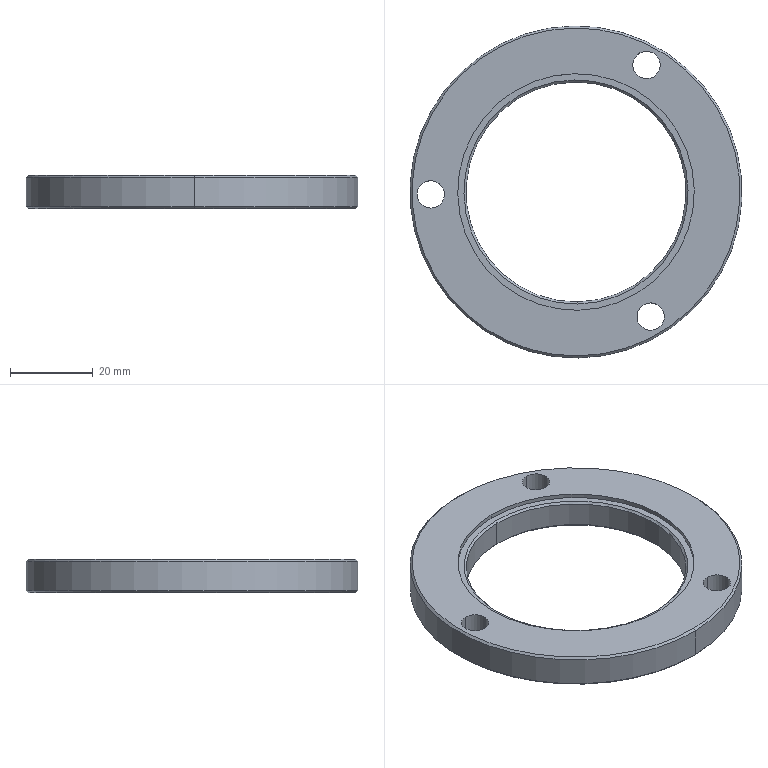Component | SolidWorks | 8TC-A17001-20-08BearingCap-1 | 1 solid | 23 faces | box 80 x 80 x 8 mm | volume 21292 mm3 | cylinder 12 | cone 8 | plane 3 | commonest cylinder face diameters 6.6 x6 57 x2 53 x2 80 x2 | material A3
STEP:
#1=COLOUR_RGB('',0.7922,0.8196,0.9333);
#2=FILL_AREA_STYLE_COLOUR('',#1);
#3=FILL_AREA_STYLE('',(#2));
#4=SURFACE_STYLE_FILL_AREA(#3);
#5=SURFACE_SIDE_STYLE('',(#4));
#6=SURFACE_STYLE_USAGE(.BOTH.,#5);
#7=PRESENTATION_STYLE_ASSIGNMENT((#6));
#8=CARTESIAN_POINT('',(28.834,9.457,-0.01969));
#9=VERTEX_POINT('',#8);
#10=CARTESIAN_POINT('',(28.885,6.348,-0.01969));
#11=VERTEX_POINT('',#10);
#12=CARTESIAN_POINT('',(28.859,7.902,-0.01969));
#13=DIRECTION('',(-0.,-0.,-1.));
#14=DIRECTION('',(0.01645,-0.9999,0.));
#15=AXIS2_PLACEMENT_3D('',#12,#13,#14);
#16=CIRCLE('',#15,1.555);
#17=EDGE_CURVE('',#9,#11,#16,.T.);
#18=ORIENTED_EDGE('',*,*,#17,.F.);
#19=CARTESIAN_POINT('',(28.833,9.477,0.));
#20=VERTEX_POINT('',#19);
#21=CARTESIAN_POINT('',(28.833,9.477,0.));
#22=DIRECTION('',(-0.01163,0.707,0.7071));
#23=VECTOR('',#22,39.37);
#24=LINE('',#21,#23);
#25=EDGE_CURVE('',#9,#20,#24,.T.);
#26=ORIENTED_EDGE('',*,*,#25,.T.);
#27=CARTESIAN_POINT('',(28.885,6.328,0.));
#28=VERTEX_POINT('',#27);
#29=CARTESIAN_POINT('',(28.859,7.902,0.));
#30=DIRECTION('',(0.,0.,1.));
#31=DIRECTION('',(0.01645,-0.9999,0.));
#32=AXIS2_PLACEMENT_3D('',#29,#30,#31);
#33=CIRCLE('',#32,1.575);
#34=EDGE_CURVE('',#28,#20,#33,.T.);
#35=ORIENTED_EDGE('',*,*,#34,.F.);
#36=CARTESIAN_POINT('',(28.885,6.328,0.));
#37=DIRECTION('',(0.01163,-0.707,0.7071));
#38=VECTOR('',#37,39.37);
#39=LINE('',#36,#38);
#40=EDGE_CURVE('',#11,#28,#39,.T.);
#41=ORIENTED_EDGE('',*,*,#40,.F.);
#42=EDGE_LOOP('',(#18,#26,#35,#41));
#43=FACE_OUTER_BOUND('',#42,.T.);
#44=CARTESIAN_POINT('',(28.859,7.902,0.));
#45=DIRECTION('',(0.,0.,1.));
#46=DIRECTION('',(0.01645,-0.9999,0.));
#47=AXIS2_PLACEMENT_3D('',#44,#45,#46);
#48=CONICAL_SURFACE('',#47,1.575,0.7854);
#49=ADVANCED_FACE('',(#43),#48,.T.);
#50=CARTESIAN_POINT('',(28.885,6.348,0.2953));
#51=VERTEX_POINT('',#50);
#52=CARTESIAN_POINT('',(28.834,9.457,0.2953));
#53=VERTEX_POINT('',#52);
#54=CARTESIAN_POINT('',(28.859,7.902,0.2953));
#55=DIRECTION('',(0.,0.,1.));
#56=DIRECTION('',(0.01645,-0.9999,0.));
#57=AXIS2_PLACEMENT_3D('',#54,#55,#56);
#58=CIRCLE('',#57,1.555);
#59=EDGE_CURVE('',#51,#53,#58,.T.);
#60=ORIENTED_EDGE('',*,*,#59,.F.);
#61=CARTESIAN_POINT('',(28.885,6.328,0.2756));
#62=VERTEX_POINT('',#61);
#63=CARTESIAN_POINT('',(28.885,6.348,0.2953));
#64=DIRECTION('',(0.01163,-0.707,-0.7071));
#65=VECTOR('',#64,39.37);
#66=LINE('',#63,#65);
#67=EDGE_CURVE('',#51,#62,#66,.T.);
#68=ORIENTED_EDGE('',*,*,#67,.T.);
#69=CARTESIAN_POINT('',(28.833,9.477,0.2756));
#70=VERTEX_POINT('',#69);
#71=CARTESIAN_POINT('',(28.859,7.902,0.2756));
#72=DIRECTION('',(-0.,-0.,-1.));
#73=DIRECTION('',(0.01645,-0.9999,0.));
#74=AXIS2_PLACEMENT_3D('',#71,#72,#73);
#75=CIRCLE('',#74,1.575);
#76=EDGE_CURVE('',#70,#62,#75,.T.);
#77=ORIENTED_EDGE('',*,*,#76,.F.);
#78=CARTESIAN_POINT('',(28.834,9.457,0.2953));
#79=DIRECTION('',(-0.01163,0.707,-0.7071));
#80=VECTOR('',#79,39.37);
#81=LINE('',#78,#80);
#82=EDGE_CURVE('',#53,#70,#81,.T.);
#83=ORIENTED_EDGE('',*,*,#82,.F.);
#84=EDGE_LOOP('',(#60,#68,#77,#83));
#85=FACE_OUTER_BOUND('',#84,.T.);
#86=CARTESIAN_POINT('',(28.859,7.902,0.2953));
#87=DIRECTION('',(-0.,-0.,-1.));
#88=DIRECTION('',(-0.01645,0.9999,0.));
#89=AXIS2_PLACEMENT_3D('',#86,#87,#88);
#90=CONICAL_SURFACE('',#89,1.555,0.7854);
#91=ADVANCED_FACE('',(#85),#90,.T.);
#92=CARTESIAN_POINT('',(28.842,8.946,0.2362));
#93=VERTEX_POINT('',#92);
#94=CARTESIAN_POINT('',(28.877,6.859,0.2362));
#95=VERTEX_POINT('',#94);
#96=CARTESIAN_POINT('',(28.859,7.902,0.2362));
#97=DIRECTION('',(0.,0.,1.));
#98=DIRECTION('',(-0.01645,0.9999,0.));
#99=AXIS2_PLACEMENT_3D('',#96,#97,#98);
#100=CIRCLE('',#99,1.043);
#101=EDGE_CURVE('',#93,#95,#100,.T.);
#102=ORIENTED_EDGE('',*,*,#101,.F.);
#103=CARTESIAN_POINT('',(28.842,8.965,0.2559));
#104=VERTEX_POINT('',#103);
#105=CARTESIAN_POINT('',(28.842,8.965,0.2559));
#106=DIRECTION('',(-0.01163,0.707,0.7071));
#107=VECTOR('',#106,39.37);
#108=LINE('',#105,#107);
#109=EDGE_CURVE('',#93,#104,#108,.T.);
#110=ORIENTED_EDGE('',*,*,#109,.T.);
#111=CARTESIAN_POINT('',(28.877,6.84,0.2559));
#112=VERTEX_POINT('',#111);
#113=CARTESIAN_POINT('',(28.859,7.902,0.2559));
#114=DIRECTION('',(-0.,-0.,-1.));
#115=DIRECTION('',(-0.01645,0.9999,0.));
#116=AXIS2_PLACEMENT_3D('',#113,#114,#115);
#117=CIRCLE('',#116,1.063);
#118=EDGE_CURVE('',#112,#104,#117,.T.);
#119=ORIENTED_EDGE('',*,*,#118,.F.);
#120=CARTESIAN_POINT('',(28.877,6.84,0.2559));
#121=DIRECTION('',(0.01163,-0.707,0.7071));
#122=VECTOR('',#121,39.37);
#123=LINE('',#120,#122);
#124=EDGE_CURVE('',#95,#112,#123,.T.);
#125=ORIENTED_EDGE('',*,*,#124,.F.);
#126=EDGE_LOOP('',(#102,#110,#119,#125));
#127=FACE_OUTER_BOUND('',#126,.T.);
#128=CARTESIAN_POINT('',(28.859,7.902,0.2559));
#129=DIRECTION('',(0.,0.,1.));
#130=DIRECTION('',(0.01645,-0.9999,0.));
#131=AXIS2_PLACEMENT_3D('',#128,#129,#130);
#132=CONICAL_SURFACE('',#131,1.063,0.7854);
#133=ADVANCED_FACE('',(#127),#132,.F.);
#134=CARTESIAN_POINT('',(28.877,6.859,0.));
#135=VERTEX_POINT('',#134);
#136=CARTESIAN_POINT('',(28.842,8.946,0.));
#137=VERTEX_POINT('',#136);
#138=CARTESIAN_POINT('',(28.859,7.902,0.));
#139=DIRECTION('',(-0.,-0.,-1.));
#140=DIRECTION('',(0.01645,-0.9999,0.));
#141=AXIS2_PLACEMENT_3D('',#138,#139,#140);
#142=CIRCLE('',#141,1.043);
#143=EDGE_CURVE('',#135,#137,#142,.T.);
#144=ORIENTED_EDGE('',*,*,#143,.F.);
#145=CARTESIAN_POINT('',(28.877,6.84,-0.01969));
#146=VERTEX_POINT('',#145);
#147=CARTESIAN_POINT('',(28.877,6.84,-0.01969));
#148=DIRECTION('',(0.01163,-0.707,-0.7071));
#149=VECTOR('',#148,39.37);
#150=LINE('',#147,#149);
#151=EDGE_CURVE('',#135,#146,#150,.T.);
#152=ORIENTED_EDGE('',*,*,#151,.T.);
#153=CARTESIAN_POINT('',(28.842,8.965,-0.01969));
#154=VERTEX_POINT('',#153);
#155=CARTESIAN_POINT('',(28.859,7.902,-0.01969));
#156=DIRECTION('',(0.,0.,1.));
#157=DIRECTION('',(0.01645,-0.9999,0.));
#158=AXIS2_PLACEMENT_3D('',#155,#156,#157);
#159=CIRCLE('',#158,1.063);
#160=EDGE_CURVE('',#154,#146,#159,.T.);
#161=ORIENTED_EDGE('',*,*,#160,.F.);
#162=CARTESIAN_POINT('',(28.842,8.965,-0.01969));
#163=DIRECTION('',(-0.01163,0.707,-0.7071));
#164=VECTOR('',#163,39.37);
#165=LINE('',#162,#164);
#166=EDGE_CURVE('',#137,#154,#165,.T.);
#167=ORIENTED_EDGE('',*,*,#166,.F.);
#168=EDGE_LOOP('',(#144,#152,#161,#167));
#169=FACE_OUTER_BOUND('',#168,.T.);
#170=CARTESIAN_POINT('',(28.859,7.902,-0.01969));
#171=DIRECTION('',(-0.,-0.,-1.));
#172=DIRECTION('',(-0.01645,0.9999,0.));
#173=AXIS2_PLACEMENT_3D('',#170,#171,#172);
#174=CONICAL_SURFACE('',#173,1.063,0.7854);
#175=ADVANCED_FACE('',(#169),#174,.F.);
#176=CARTESIAN_POINT('',(29.57,6.591,0.2953));
#177=VERTEX_POINT('',#176);
#178=CARTESIAN_POINT('',(29.566,6.85,0.2953));
#179=VERTEX_POINT('',#178);
#180=CARTESIAN_POINT('',(29.568,6.721,0.2953));
#181=DIRECTION('',(-0.,-0.,-1.));
#182=DIRECTION('',(-0.01645,0.9999,0.));
#183=AXIS2_PLACEMENT_3D('',#180,#181,#182);
#184=CIRCLE('',#183,0.1299);
#185=EDGE_CURVE('',#177,#179,#184,.T.);
#186=ORIENTED_EDGE('',*,*,#185,.F.);
#187=CARTESIAN_POINT('',(29.57,6.591,-0.01969));
#188=VERTEX_POINT('',#187);
#189=CARTESIAN_POINT('',(29.57,6.591,-0.01969));
#190=DIRECTION('',(-0.,-0.,-1.));
#191=VECTOR('',#190,39.37);
#192=LINE('',#189,#191);
#193=EDGE_CURVE('',#177,#188,#192,.T.);
#194=ORIENTED_EDGE('',*,*,#193,.T.);
#195=CARTESIAN_POINT('',(29.566,6.85,-0.01969));
#196=VERTEX_POINT('',#195);
#197=CARTESIAN_POINT('',(29.568,6.721,-0.01969));
#198=DIRECTION('',(-0.,-0.,-1.));
#199=DIRECTION('',(-0.01645,0.9999,0.));
#200=AXIS2_PLACEMENT_3D('',#197,#198,#199);
#201=CIRCLE('',#200,0.1299);
#202=EDGE_CURVE('',#188,#196,#201,.T.);
#203=ORIENTED_EDGE('',*,*,#202,.T.);
#204=CARTESIAN_POINT('',(29.566,6.85,-0.01969));
#205=DIRECTION('',(-0.,-0.,-1.));
#206=VECTOR('',#205,39.37);
#207=LINE('',#204,#206);
#208=EDGE_CURVE('',#179,#196,#207,.T.);
#209=ORIENTED_EDGE('',*,*,#208,.F.);
#210=EDGE_LOOP('',(#186,#194,#203,#209));
#211=FACE_OUTER_BOUND('',#210,.T.);
#212=CARTESIAN_POINT('',(29.568,6.721,-0.01969));
#213=DIRECTION('',(-0.,-0.,-1.));
#214=DIRECTION('',(-0.01645,0.9999,0.));
#215=AXIS2_PLACEMENT_3D('',#212,#213,#214);
#216=CYLINDRICAL_SURFACE('',#215,0.1299);
#217=ADVANCED_FACE('',(#211),#216,.F.);
#218=CARTESIAN_POINT('',(29.531,8.977,0.2953));
#219=VERTEX_POINT('',#218);
#220=CARTESIAN_POINT('',(29.527,9.237,0.2953));
#221=VERTEX_POINT('',#220);
#222=CARTESIAN_POINT('',(29.529,9.107,0.2953));
#223=DIRECTION('',(-0.,-0.,-1.));
#224=DIRECTION('',(-0.01645,0.9999,0.));
#225=AXIS2_PLACEMENT_3D('',#222,#223,#224);
#226=CIRCLE('',#225,0.1299);
#227=EDGE_CURVE('',#219,#221,#226,.T.);
#228=ORIENTED_EDGE('',*,*,#227,.F.);
#229=CARTESIAN_POINT('',(29.531,8.977,-0.01969));
#230=VERTEX_POINT('',#229);
#231=CARTESIAN_POINT('',(29.531,8.977,-0.01969));
#232=DIRECTION('',(-0.,-0.,-1.));
#233=VECTOR('',#232,39.37);
#234=LINE('',#231,#233);
#235=EDGE_CURVE('',#219,#230,#234,.T.);
#236=ORIENTED_EDGE('',*,*,#235,.T.);
#237=CARTESIAN_POINT('',(29.527,9.237,-0.01969));
#238=VERTEX_POINT('',#237);
#239=CARTESIAN_POINT('',(29.529,9.107,-0.01969));
#240=DIRECTION('',(-0.,-0.,-1.));
#241=DIRECTION('',(-0.01645,0.9999,0.));
#242=AXIS2_PLACEMENT_3D('',#239,#240,#241);
#243=CIRCLE('',#242,0.1299);
#244=EDGE_CURVE('',#230,#238,#243,.T.);
#245=ORIENTED_EDGE('',*,*,#244,.T.);
#246=CARTESIAN_POINT('',(29.527,9.237,-0.01969));
#247=DIRECTION('',(-0.,-0.,-1.));
#248=VECTOR('',#247,39.37);
#249=LINE('',#246,#248);
#250=EDGE_CURVE('',#221,#238,#249,.T.);
#251=ORIENTED_EDGE('',*,*,#250,.F.);
#252=EDGE_LOOP('',(#228,#236,#245,#251));
#253=FACE_OUTER_BOUND('',#252,.T.);
#254=CARTESIAN_POINT('',(29.529,9.107,-0.01969));
#255=DIRECTION('',(-0.,-0.,-1.));
#256=DIRECTION('',(-0.01645,0.9999,0.));
#257=AXIS2_PLACEMENT_3D('',#254,#255,#256);
#258=CYLINDRICAL_SURFACE('',#257,0.1299);
#259=ADVANCED_FACE('',(#253),#258,.F.);
#260=CARTESIAN_POINT('',(27.484,7.75,0.2953));
#261=VERTEX_POINT('',#260);
#262=CARTESIAN_POINT('',(27.479,8.01,0.2953));
#263=VERTEX_POINT('',#262);
#264=CARTESIAN_POINT('',(27.482,7.88,0.2953));
#265=DIRECTION('',(-0.,-0.,-1.));
#266=DIRECTION('',(-0.01645,0.9999,0.));
#267=AXIS2_PLACEMENT_3D('',#264,#265,#266);
#268=CIRCLE('',#267,0.1299);
#269=EDGE_CURVE('',#261,#263,#268,.T.);
#270=ORIENTED_EDGE('',*,*,#269,.F.);
#271=CARTESIAN_POINT('',(27.484,7.75,-0.01969));
#272=VERTEX_POINT('',#271);
#273=CARTESIAN_POINT('',(27.484,7.75,-0.01969));
#274=DIRECTION('',(-0.,-0.,-1.));
#275=VECTOR('',#274,39.37);
#276=LINE('',#273,#275);
#277=EDGE_CURVE('',#261,#272,#276,.T.);
#278=ORIENTED_EDGE('',*,*,#277,.T.);
#279=CARTESIAN_POINT('',(27.479,8.01,-0.01969));
#280=VERTEX_POINT('',#279);
#281=CARTESIAN_POINT('',(27.482,7.88,-0.01969));
#282=DIRECTION('',(-0.,-0.,-1.));
#283=DIRECTION('',(-0.01645,0.9999,0.));
#284=AXIS2_PLACEMENT_3D('',#281,#282,#283);
#285=CIRCLE('',#284,0.1299);
#286=EDGE_CURVE('',#272,#280,#285,.T.);
#287=ORIENTED_EDGE('',*,*,#286,.T.);
#288=CARTESIAN_POINT('',(27.479,8.01,-0.01969));
#289=DIRECTION('',(-0.,-0.,-1.));
#290=VECTOR('',#289,39.37);
#291=LINE('',#288,#290);
#292=EDGE_CURVE('',#263,#280,#291,.T.);
#293=ORIENTED_EDGE('',*,*,#292,.F.);
#294=EDGE_LOOP('',(#270,#278,#287,#293));
#295=FACE_OUTER_BOUND('',#294,.T.);
#296=CARTESIAN_POINT('',(27.482,7.88,-0.01969));
#297=DIRECTION('',(-0.,-0.,-1.));
#298=DIRECTION('',(-0.01645,0.9999,0.));
#299=AXIS2_PLACEMENT_3D('',#296,#297,#298);
#300=CYLINDRICAL_SURFACE('',#299,0.1299);
#301=ADVANCED_FACE('',(#295),#300,.F.);
#302=CARTESIAN_POINT('',(28.878,6.781,0.2559));
#303=VERTEX_POINT('',#302);
#304=CARTESIAN_POINT('',(28.841,9.024,0.2559));
#305=VERTEX_POINT('',#304);
#306=CARTESIAN_POINT('',(28.859,7.902,0.2559));
#307=DIRECTION('',(-0.,-0.,-1.));
#308=DIRECTION('',(-0.01645,0.9999,0.));
#309=AXIS2_PLACEMENT_3D('',#306,#307,#308);
#310=CIRCLE('',#309,1.122);
#311=EDGE_CURVE('',#303,#305,#310,.T.);
#312=ORIENTED_EDGE('',*,*,#311,.T.);
#313=CARTESIAN_POINT('',(28.841,9.024,0.2953));
#314=VERTEX_POINT('',#313);
#315=CARTESIAN_POINT('',(28.841,9.024,0.2559));
#316=DIRECTION('',(0.,0.,1.));
#317=VECTOR('',#316,39.37);
#318=LINE('',#315,#317);
#319=EDGE_CURVE('',#305,#314,#318,.T.);
#320=ORIENTED_EDGE('',*,*,#319,.T.);
#321=CARTESIAN_POINT('',(28.878,6.781,0.2953));
#322=VERTEX_POINT('',#321);
#323=CARTESIAN_POINT('',(28.859,7.902,0.2953));
#324=DIRECTION('',(-0.,-0.,-1.));
#325=DIRECTION('',(-0.01645,0.9999,0.));
#326=AXIS2_PLACEMENT_3D('',#323,#324,#325);
#327=CIRCLE('',#326,1.122);
#328=EDGE_CURVE('',#322,#314,#327,.T.);
#329=ORIENTED_EDGE('',*,*,#328,.F.);
#330=CARTESIAN_POINT('',(28.878,6.781,0.2559));
#331=DIRECTION('',(0.,0.,1.));
#332=VECTOR('',#331,39.37);
#333=LINE('',#330,#332);
#334=EDGE_CURVE('',#303,#322,#333,.T.);
#335=ORIENTED_EDGE('',*,*,#334,.F.);
#336=EDGE_LOOP('',(#312,#320,#329,#335));
#337=FACE_OUTER_BOUND('',#336,.T.);
#338=CARTESIAN_POINT('',(28.859,7.902,0.2559));
#339=DIRECTION('',(0.,0.,1.));
#340=DIRECTION('',(0.01645,-0.9999,0.));
#341=AXIS2_PLACEMENT_3D('',#338,#339,#340);
#342=CYLINDRICAL_SURFACE('',#341,1.122);
#343=ADVANCED_FACE('',(#337),#342,.F.);
#344=ORIENTED_EDGE('',*,*,#101,.T.);
#345=CARTESIAN_POINT('',(28.877,6.859,0.2953));
#346=DIRECTION('',(-0.,-0.,-1.));
#347=VECTOR('',#346,39.37);
#348=LINE('',#345,#347);
#349=EDGE_CURVE('',#95,#135,#348,.T.);
#350=ORIENTED_EDGE('',*,*,#349,.T.);
#351=ORIENTED_EDGE('',*,*,#143,.T.);
#352=CARTESIAN_POINT('',(28.842,8.946,0.2953));
#353=DIRECTION('',(-0.,-0.,-1.));
#354=VECTOR('',#353,39.37);
#355=LINE('',#352,#354);
#356=EDGE_CURVE('',#93,#137,#355,.T.);
#357=ORIENTED_EDGE('',*,*,#356,.F.);
#358=EDGE_LOOP('',(#344,#350,#351,#357));
#359=FACE_OUTER_BOUND('',#358,.T.);
#360=CARTESIAN_POINT('',(28.859,7.902,0.2953));
#361=DIRECTION('',(-0.,-0.,-1.));
#362=DIRECTION('',(-0.01645,0.9999,0.));
#363=AXIS2_PLACEMENT_3D('',#360,#361,#362);
#364=CYLINDRICAL_SURFACE('',#363,1.043);
#365=ADVANCED_FACE('',(#359),#364,.F.);
#366=ORIENTED_EDGE('',*,*,#76,.T.);
#367=CARTESIAN_POINT('',(28.885,6.328,0.2953));
#368=DIRECTION('',(-0.,-0.,-1.));
#369=VECTOR('',#368,39.37);
#370=LINE('',#367,#369);
#371=EDGE_CURVE('',#62,#28,#370,.T.);
#372=ORIENTED_EDGE('',*,*,#371,.T.);
#373=ORIENTED_EDGE('',*,*,#34,.T.);
#374=CARTESIAN_POINT('',(28.833,9.477,0.2953));
#375=DIRECTION('',(-0.,-0.,-1.));
#376=VECTOR('',#375,39.37);
#377=LINE('',#374,#376);
#378=EDGE_CURVE('',#70,#20,#377,.T.);
#379=ORIENTED_EDGE('',*,*,#378,.F.);
#380=EDGE_LOOP('',(#366,#372,#373,#379));
#381=FACE_OUTER_BOUND('',#380,.T.);
#382=CARTESIAN_POINT('',(28.859,7.902,0.2953));
#383=DIRECTION('',(-0.,-0.,-1.));
#384=DIRECTION('',(-0.01645,0.9999,0.));
#385=AXIS2_PLACEMENT_3D('',#382,#383,#384);
#386=CYLINDRICAL_SURFACE('',#385,1.575);
#387=ADVANCED_FACE('',(#381),#386,.T.);
#388=CARTESIAN_POINT('',(28.859,7.902,0.2953));
#389=DIRECTION('',(0.,0.,1.));
#390=DIRECTION('',(0.01645,-0.9999,0.));
#391=AXIS2_PLACEMENT_3D('',#388,#389,#390);
#392=CIRCLE('',#391,1.555);
#393=EDGE_CURVE('',#53,#51,#392,.T.);
#394=ORIENTED_EDGE('',*,*,#393,.T.);
#395=ORIENTED_EDGE('',*,*,#59,.T.);
#396=EDGE_LOOP('',(#394,#395));
#397=FACE_OUTER_BOUND('',#396,.T.);
#398=CARTESIAN_POINT('',(29.568,6.721,0.2953));
#399=DIRECTION('',(-0.,-0.,-1.));
#400=DIRECTION('',(-0.01645,0.9999,0.));
#401=AXIS2_PLACEMENT_3D('',#398,#399,#400);
#402=CIRCLE('',#401,0.1299);
#403=EDGE_CURVE('',#179,#177,#402,.T.);
#404=ORIENTED_EDGE('',*,*,#403,.T.);
#405=ORIENTED_EDGE('',*,*,#185,.T.);
#406=EDGE_LOOP('',(#404,#405));
#407=FACE_BOUND('',#406,.T.);
#408=CARTESIAN_POINT('',(29.529,9.107,0.2953));
#409=DIRECTION('',(-0.,-0.,-1.));
#410=DIRECTION('',(-0.01645,0.9999,0.));
#411=AXIS2_PLACEMENT_3D('',#408,#409,#410);
#412=CIRCLE('',#411,0.1299);
#413=EDGE_CURVE('',#221,#219,#412,.T.);
#414=ORIENTED_EDGE('',*,*,#413,.T.);
#415=ORIENTED_EDGE('',*,*,#227,.T.);
#416=EDGE_LOOP('',(#414,#415));
#417=FACE_BOUND('',#416,.T.);
#418=CARTESIAN_POINT('',(27.482,7.88,0.2953));
#419=DIRECTION('',(-0.,-0.,-1.));
#420=DIRECTION('',(-0.01645,0.9999,0.));
#421=AXIS2_PLACEMENT_3D('',#418,#419,#420);
#422=CIRCLE('',#421,0.1299);
#423=EDGE_CURVE('',#263,#261,#422,.T.);
#424=ORIENTED_EDGE('',*,*,#423,.T.);
#425=ORIENTED_EDGE('',*,*,#269,.T.);
#426=EDGE_LOOP('',(#424,#425));
#427=FACE_BOUND('',#426,.T.);
#428=ORIENTED_EDGE('',*,*,#328,.T.);
#429=CARTESIAN_POINT('',(28.859,7.902,0.2953));
#430=DIRECTION('',(-0.,-0.,-1.));
#431=DIRECTION('',(-0.01645,0.9999,0.));
#432=AXIS2_PLACEMENT_3D('',#429,#430,#431);
#433=CIRCLE('',#432,1.122);
#434=EDGE_CURVE('',#314,#322,#433,.T.);
#435=ORIENTED_EDGE('',*,*,#434,.T.);
#436=EDGE_LOOP('',(#428,#435));
#437=FACE_BOUND('',#436,.T.);
#438=CARTESIAN_POINT('',(28.859,7.902,0.2953));
#439=DIRECTION('',(0.,0.,1.));
#440=DIRECTION('',(0.01645,-0.9999,0.));
#441=AXIS2_PLACEMENT_3D('',#438,#439,#440);
#442=PLANE('',#441);
#443=ADVANCED_FACE('',(#397,#407,#417,#427,#437),#442,.T.);
#444=ORIENTED_EDGE('',*,*,#160,.T.);
#445=CARTESIAN_POINT('',(28.859,7.902,-0.01969));
#446=DIRECTION('',(0.,0.,1.));
#447=DIRECTION('',(0.01645,-0.9999,0.));
#448=AXIS2_PLACEMENT_3D('',#445,#446,#447);
#449=CIRCLE('',#448,1.063);
#450=EDGE_CURVE('',#146,#154,#449,.T.);
#451=ORIENTED_EDGE('',*,*,#450,.T.);
#452=EDGE_LOOP('',(#444,#451));
#453=FACE_BOUND('',#452,.T.);
#454=CARTESIAN_POINT('',(28.859,7.902,-0.01969));
#455=DIRECTION('',(-0.,-0.,-1.));
#456=DIRECTION('',(0.01645,-0.9999,0.));
#457=AXIS2_PLACEMENT_3D('',#454,#455,#456);
#458=CIRCLE('',#457,1.555);
#459=EDGE_CURVE('',#11,#9,#458,.T.);
#460=ORIENTED_EDGE('',*,*,#459,.T.);
#461=ORIENTED_EDGE('',*,*,#17,.T.);
#462=EDGE_LOOP('',(#460,#461));
#463=FACE_OUTER_BOUND('',#462,.T.);
#464=CARTESIAN_POINT('',(29.568,6.721,-0.01969));
#465=DIRECTION('',(-0.,-0.,-1.));
#466=DIRECTION('',(-0.01645,0.9999,0.));
#467=AXIS2_PLACEMENT_3D('',#464,#465,#466);
#468=CIRCLE('',#467,0.1299);
#469=EDGE_CURVE('',#196,#188,#468,.T.);
#470=ORIENTED_EDGE('',*,*,#469,.F.);
#471=ORIENTED_EDGE('',*,*,#202,.F.);
#472=EDGE_LOOP('',(#470,#471));
#473=FACE_BOUND('',#472,.T.);
#474=CARTESIAN_POINT('',(29.529,9.107,-0.01969));
#475=DIRECTION('',(-0.,-0.,-1.));
#476=DIRECTION('',(-0.01645,0.9999,0.));
#477=AXIS2_PLACEMENT_3D('',#474,#475,#476);
#478=CIRCLE('',#477,0.1299);
#479=EDGE_CURVE('',#238,#230,#478,.T.);
#480=ORIENTED_EDGE('',*,*,#479,.F.);
#481=ORIENTED_EDGE('',*,*,#244,.F.);
#482=EDGE_LOOP('',(#480,#481));
#483=FACE_BOUND('',#482,.T.);
#484=CARTESIAN_POINT('',(27.482,7.88,-0.01969));
#485=DIRECTION('',(-0.,-0.,-1.));
#486=DIRECTION('',(-0.01645,0.9999,0.));
#487=AXIS2_PLACEMENT_3D('',#484,#485,#486);
#488=CIRCLE('',#487,0.1299);
#489=EDGE_CURVE('',#280,#272,#488,.T.);
#490=ORIENTED_EDGE('',*,*,#489,.F.);
#491=ORIENTED_EDGE('',*,*,#286,.F.);
#492=EDGE_LOOP('',(#490,#491));
#493=FACE_BOUND('',#492,.T.);
#494=CARTESIAN_POINT('',(28.859,7.902,-0.01969));
#495=DIRECTION('',(0.,0.,1.));
#496=DIRECTION('',(0.01645,-0.9999,0.));
#497=AXIS2_PLACEMENT_3D('',#494,#495,#496);
#498=PLANE('',#497);
#499=ADVANCED_FACE('',(#453,#463,#473,#483,#493),#498,.F.);
#500=ORIENTED_EDGE('',*,*,#371,.F.);
#501=CARTESIAN_POINT('',(28.859,7.902,0.2756));
#502=DIRECTION('',(-0.,-0.,-1.));
#503=DIRECTION('',(0.01645,-0.9999,0.));
#504=AXIS2_PLACEMENT_3D('',#501,#502,#503);
#505=CIRCLE('',#504,1.575);
#506=EDGE_CURVE('',#62,#70,#505,.T.);
#507=ORIENTED_EDGE('',*,*,#506,.T.);
#508=ORIENTED_EDGE('',*,*,#378,.T.);
#509=CARTESIAN_POINT('',(28.859,7.902,0.));
#510=DIRECTION('',(0.,0.,1.));
#511=DIRECTION('',(0.01645,-0.9999,0.));
#512=AXIS2_PLACEMENT_3D('',#509,#510,#511);
#513=CIRCLE('',#512,1.575);
#514=EDGE_CURVE('',#20,#28,#513,.T.);
#515=ORIENTED_EDGE('',*,*,#514,.T.);
#516=EDGE_LOOP('',(#500,#507,#508,#515));
#517=FACE_OUTER_BOUND('',#516,.T.);
#518=CARTESIAN_POINT('',(28.859,7.902,0.2953));
#519=DIRECTION('',(-0.,-0.,-1.));
#520=DIRECTION('',(-0.01645,0.9999,0.));
#521=AXIS2_PLACEMENT_3D('',#518,#519,#520);
#522=CYLINDRICAL_SURFACE('',#521,1.575);
#523=ADVANCED_FACE('',(#517),#522,.T.);
#524=ORIENTED_EDGE('',*,*,#349,.F.);
#525=CARTESIAN_POINT('',(28.859,7.902,0.2362));
#526=DIRECTION('',(0.,0.,1.));
#527=DIRECTION('',(-0.01645,0.9999,0.));
#528=AXIS2_PLACEMENT_3D('',#525,#526,#527);
#529=CIRCLE('',#528,1.043);
#530=EDGE_CURVE('',#95,#93,#529,.T.);
#531=ORIENTED_EDGE('',*,*,#530,.T.);
#532=ORIENTED_EDGE('',*,*,#356,.T.);
#533=CARTESIAN_POINT('',(28.859,7.902,0.));
#534=DIRECTION('',(-0.,-0.,-1.));
#535=DIRECTION('',(0.01645,-0.9999,0.));
#536=AXIS2_PLACEMENT_3D('',#533,#534,#535);
#537=CIRCLE('',#536,1.043);
#538=EDGE_CURVE('',#137,#135,#537,.T.);
#539=ORIENTED_EDGE('',*,*,#538,.T.);
#540=EDGE_LOOP('',(#524,#531,#532,#539));
#541=FACE_OUTER_BOUND('',#540,.T.);
#542=CARTESIAN_POINT('',(28.859,7.902,0.2953));
#543=DIRECTION('',(-0.,-0.,-1.));
#544=DIRECTION('',(-0.01645,0.9999,0.));
#545=AXIS2_PLACEMENT_3D('',#542,#543,#544);
#546=CYLINDRICAL_SURFACE('',#545,1.043);
#547=ADVANCED_FACE('',(#541),#546,.F.);
#548=ORIENTED_EDGE('',*,*,#319,.F.);
#549=CARTESIAN_POINT('',(28.859,7.902,0.2559));
#550=DIRECTION('',(-0.,-0.,-1.));
#551=DIRECTION('',(-0.01645,0.9999,0.));
#552=AXIS2_PLACEMENT_3D('',#549,#550,#551);
#553=CIRCLE('',#552,1.122);
#554=EDGE_CURVE('',#305,#303,#553,.T.);
#555=ORIENTED_EDGE('',*,*,#554,.T.);
#556=ORIENTED_EDGE('',*,*,#334,.T.);
#557=ORIENTED_EDGE('',*,*,#434,.F.);
#558=EDGE_LOOP('',(#548,#555,#556,#557));
#559=FACE_OUTER_BOUND('',#558,.T.);
#560=CARTESIAN_POINT('',(28.859,7.902,0.2559));
#561=DIRECTION('',(0.,0.,1.));
#562=DIRECTION('',(0.01645,-0.9999,0.));
#563=AXIS2_PLACEMENT_3D('',#560,#561,#562);
#564=CYLINDRICAL_SURFACE('',#563,1.122);
#565=ADVANCED_FACE('',(#559),#564,.F.);
#566=ORIENTED_EDGE('',*,*,#118,.T.);
#567=CARTESIAN_POINT('',(28.859,7.902,0.2559));
#568=DIRECTION('',(-0.,-0.,-1.));
#569=DIRECTION('',(-0.01645,0.9999,0.));
#570=AXIS2_PLACEMENT_3D('',#567,#568,#569);
#571=CIRCLE('',#570,1.063);
#572=EDGE_CURVE('',#104,#112,#571,.T.);
#573=ORIENTED_EDGE('',*,*,#572,.T.);
#574=EDGE_LOOP('',(#566,#573));
#575=FACE_BOUND('',#574,.T.);
#576=ORIENTED_EDGE('',*,*,#311,.F.);
#577=ORIENTED_EDGE('',*,*,#554,.F.);
#578=EDGE_LOOP('',(#576,#577));
#579=FACE_OUTER_BOUND('',#578,.T.);
#580=CARTESIAN_POINT('',(28.859,7.902,0.2559));
#581=DIRECTION('',(-0.,-0.,-1.));
#582=DIRECTION('',(-0.01645,0.9999,-0.));
#583=AXIS2_PLACEMENT_3D('',#580,#581,#582);
#584=PLANE('',#583);
#585=ADVANCED_FACE('',(#575,#579),#584,.F.);
#586=ORIENTED_EDGE('',*,*,#277,.F.);
#587=ORIENTED_EDGE('',*,*,#423,.F.);
#588=ORIENTED_EDGE('',*,*,#292,.T.);
#589=ORIENTED_EDGE('',*,*,#489,.T.);
#590=EDGE_LOOP('',(#586,#587,#588,#589));
#591=FACE_OUTER_BOUND('',#590,.T.);
#592=CARTESIAN_POINT('',(27.482,7.88,-0.01969));
#593=DIRECTION('',(-0.,-0.,-1.));
#594=DIRECTION('',(-0.01645,0.9999,0.));
#595=AXIS2_PLACEMENT_3D('',#592,#593,#594);
#596=CYLINDRICAL_SURFACE('',#595,0.1299);
#597=ADVANCED_FACE('',(#591),#596,.F.);
#598=ORIENTED_EDGE('',*,*,#235,.F.);
#599=ORIENTED_EDGE('',*,*,#413,.F.);
#600=ORIENTED_EDGE('',*,*,#250,.T.);
#601=ORIENTED_EDGE('',*,*,#479,.T.);
#602=EDGE_LOOP('',(#598,#599,#600,#601));
#603=FACE_OUTER_BOUND('',#602,.T.);
#604=CARTESIAN_POINT('',(29.529,9.107,-0.01969));
#605=DIRECTION('',(-0.,-0.,-1.));
#606=DIRECTION('',(-0.01645,0.9999,0.));
#607=AXIS2_PLACEMENT_3D('',#604,#605,#606);
#608=CYLINDRICAL_SURFACE('',#607,0.1299);
#609=ADVANCED_FACE('',(#603),#608,.F.);
#610=ORIENTED_EDGE('',*,*,#193,.F.);
#611=ORIENTED_EDGE('',*,*,#403,.F.);
#612=ORIENTED_EDGE('',*,*,#208,.T.);
#613=ORIENTED_EDGE('',*,*,#469,.T.);
#614=EDGE_LOOP('',(#610,#611,#612,#613));
#615=FACE_OUTER_BOUND('',#614,.T.);
#616=CARTESIAN_POINT('',(29.568,6.721,-0.01969));
#617=DIRECTION('',(-0.,-0.,-1.));
#618=DIRECTION('',(-0.01645,0.9999,0.));
#619=AXIS2_PLACEMENT_3D('',#616,#617,#618);
#620=CYLINDRICAL_SURFACE('',#619,0.1299);
#621=ADVANCED_FACE('',(#615),#620,.F.);
#622=ORIENTED_EDGE('',*,*,#151,.F.);
#623=ORIENTED_EDGE('',*,*,#538,.F.);
#624=ORIENTED_EDGE('',*,*,#166,.T.);
#625=ORIENTED_EDGE('',*,*,#450,.F.);
#626=EDGE_LOOP('',(#622,#623,#624,#625));
#627=FACE_OUTER_BOUND('',#626,.T.);
#628=CARTESIAN_POINT('',(28.859,7.902,-0.01969));
#629=DIRECTION('',(-0.,-0.,-1.));
#630=DIRECTION('',(-0.01645,0.9999,0.));
#631=AXIS2_PLACEMENT_3D('',#628,#629,#630);
#632=CONICAL_SURFACE('',#631,1.063,0.7854);
#633=ADVANCED_FACE('',(#627),#632,.F.);
#634=ORIENTED_EDGE('',*,*,#109,.F.);
#635=ORIENTED_EDGE('',*,*,#530,.F.);
#636=ORIENTED_EDGE('',*,*,#124,.T.);
#637=ORIENTED_EDGE('',*,*,#572,.F.);
#638=EDGE_LOOP('',(#634,#635,#636,#637));
#639=FACE_OUTER_BOUND('',#638,.T.);
#640=CARTESIAN_POINT('',(28.859,7.902,0.2559));
#641=DIRECTION('',(0.,0.,1.));
#642=DIRECTION('',(0.01645,-0.9999,0.));
#643=AXIS2_PLACEMENT_3D('',#640,#641,#642);
#644=CONICAL_SURFACE('',#643,1.063,0.7854);
#645=ADVANCED_FACE('',(#639),#644,.F.);
#646=ORIENTED_EDGE('',*,*,#67,.F.);
#647=ORIENTED_EDGE('',*,*,#393,.F.);
#648=ORIENTED_EDGE('',*,*,#82,.T.);
#649=ORIENTED_EDGE('',*,*,#506,.F.);
#650=EDGE_LOOP('',(#646,#647,#648,#649));
#651=FACE_OUTER_BOUND('',#650,.T.);
#652=CARTESIAN_POINT('',(28.859,7.902,0.2953));
#653=DIRECTION('',(-0.,-0.,-1.));
#654=DIRECTION('',(-0.01645,0.9999,0.));
#655=AXIS2_PLACEMENT_3D('',#652,#653,#654);
#656=CONICAL_SURFACE('',#655,1.555,0.7854);
#657=ADVANCED_FACE('',(#651),#656,.T.);
#658=ORIENTED_EDGE('',*,*,#25,.F.);
#659=ORIENTED_EDGE('',*,*,#459,.F.);
#660=ORIENTED_EDGE('',*,*,#40,.T.);
#661=ORIENTED_EDGE('',*,*,#514,.F.);
#662=EDGE_LOOP('',(#658,#659,#660,#661));
#663=FACE_OUTER_BOUND('',#662,.T.);
#664=CARTESIAN_POINT('',(28.859,7.902,0.));
#665=DIRECTION('',(0.,0.,1.));
#666=DIRECTION('',(0.01645,-0.9999,0.));
#667=AXIS2_PLACEMENT_3D('',#664,#665,#666);
#668=CONICAL_SURFACE('',#667,1.575,0.7854);
#669=ADVANCED_FACE('',(#663),#668,.T.);
#670=CLOSED_SHELL('',(#49,#91,#133,#175,#217,#259,#301,#343,#365,#387,#443,#499,#523,#547,#565,#585,#597,#609,#621,#633,#645,#657,#669));
#671=MANIFOLD_SOLID_BREP('',#670);
#672=STYLED_ITEM('',(#7),#671);
#673=(LENGTH_UNIT()NAMED_UNIT(*)SI_UNIT($,.METRE.));
#674=LENGTH_MEASURE_WITH_UNIT(LENGTH_MEASURE(0.0254),#673);
#675=DIMENSIONAL_EXPONENTS(1.,0.,0.,0.,0.,0.,0.);
#676=(CONVERSION_BASED_UNIT('',#674)LENGTH_UNIT()NAMED_UNIT(#675));
#677=UNCERTAINTY_MEASURE_WITH_UNIT(LENGTH_MEASURE(0.00001),#676,'','');
#678=(NAMED_UNIT(*)PLANE_ANGLE_UNIT()SI_UNIT($,.RADIAN.));
#679=(NAMED_UNIT(*)SI_UNIT($,.STERADIAN.)SOLID_ANGLE_UNIT());
#680=(GEOMETRIC_REPRESENTATION_CONTEXT(3)GLOBAL_UNCERTAINTY_ASSIGNED_CONTEXT((#677))GLOBAL_UNIT_ASSIGNED_CONTEXT((#676,#678,#679))REPRESENTATION_CONTEXT('',''));
#681=MECHANICAL_DESIGN_GEOMETRIC_PRESENTATION_REPRESENTATION('',(#672),#680);
#682=PRESENTATION_LAYER_ASSIGNMENT('','',(#672));
#683=CARTESIAN_POINT('',(0.,0.,0.));
#684=DIRECTION('',(0.,0.,1.));
#685=DIRECTION('',(1.,0.,0.));
#686=AXIS2_PLACEMENT_3D('',#683,#684,#685);
#687=(LENGTH_UNIT()NAMED_UNIT(*)SI_UNIT($,.METRE.));
#688=LENGTH_MEASURE_WITH_UNIT(LENGTH_MEASURE(0.0254),#687);
#689=DIMENSIONAL_EXPONENTS(1.,0.,0.,0.,0.,0.,0.);
#690=(CONVERSION_BASED_UNIT('',#688)LENGTH_UNIT()NAMED_UNIT(#689));
#691=UNCERTAINTY_MEASURE_WITH_UNIT(LENGTH_MEASURE(0.00001),#690,'','');
#692=(NAMED_UNIT(*)PLANE_ANGLE_UNIT()SI_UNIT($,.RADIAN.));
#693=(NAMED_UNIT(*)SI_UNIT($,.STERADIAN.)SOLID_ANGLE_UNIT());
#694=(GEOMETRIC_REPRESENTATION_CONTEXT(3)GLOBAL_UNCERTAINTY_ASSIGNED_CONTEXT((#691))GLOBAL_UNIT_ASSIGNED_CONTEXT((#690,#692,#693))REPRESENTATION_CONTEXT('',''));
#695=ADVANCED_BREP_SHAPE_REPRESENTATION('',(#671,#686),#694);